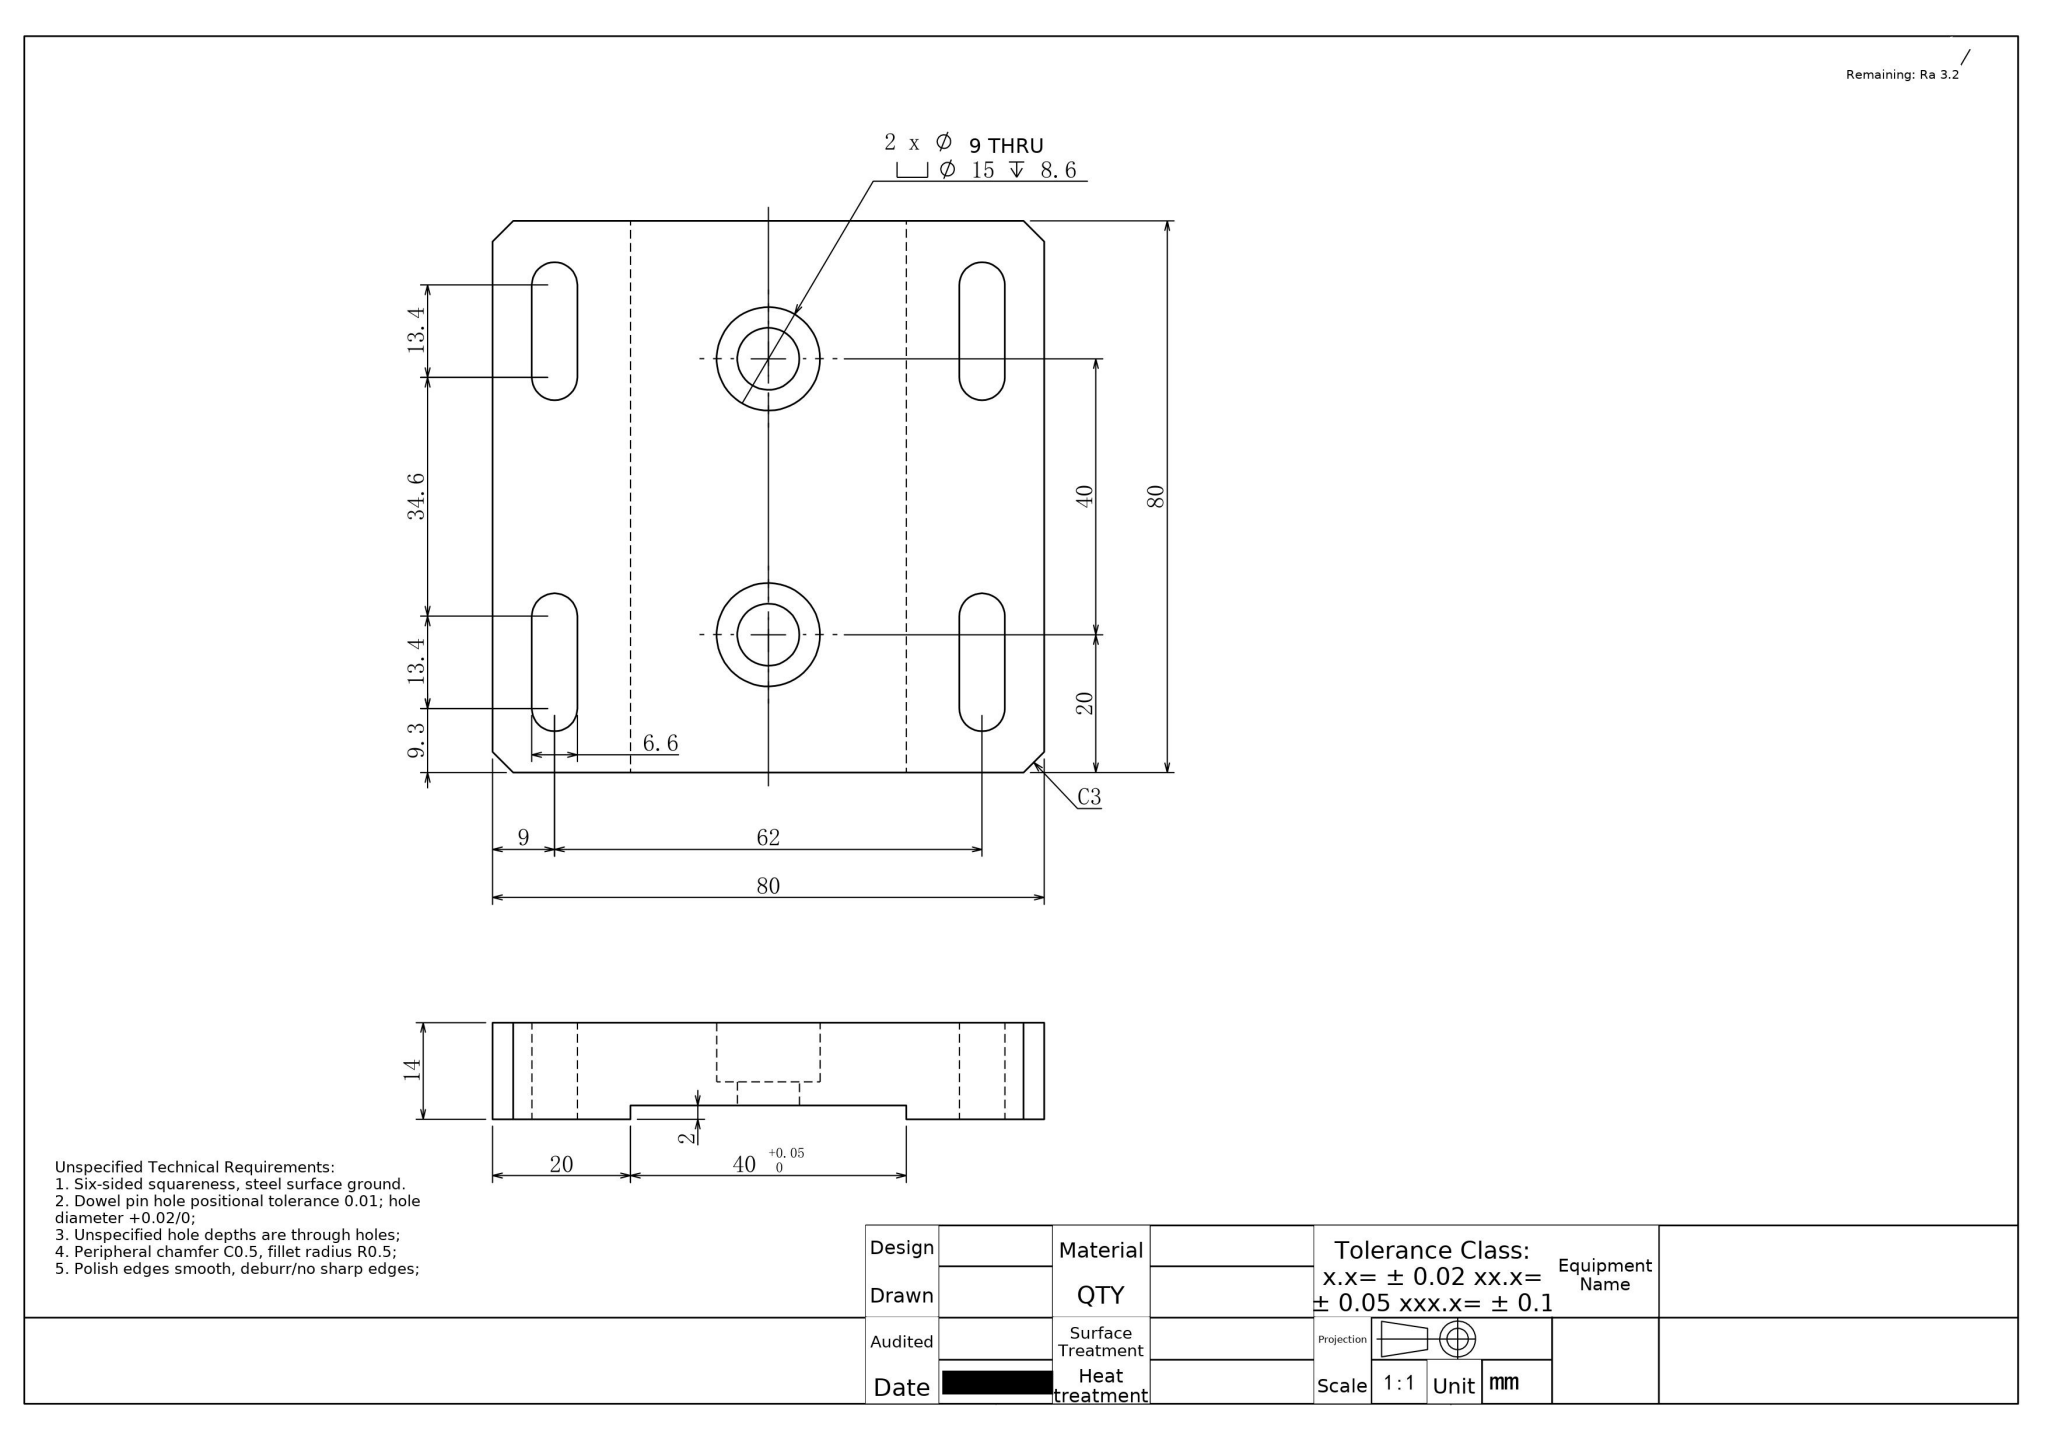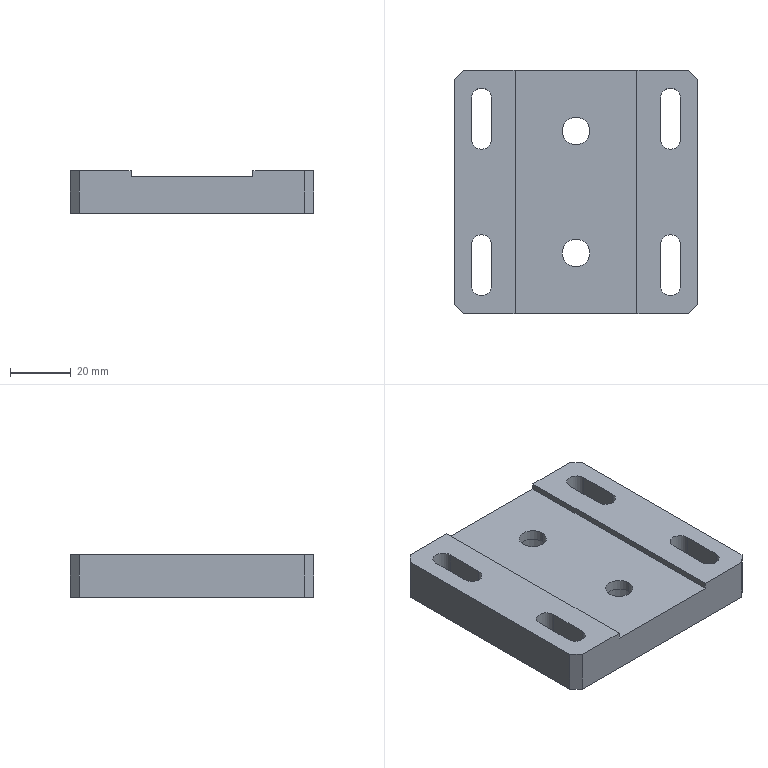Part | NX | mm | 1 solid | 40 faces | box 80 x 80 x 14 mm | volume 72607 mm3 | plane 24 | cylinder 16 | commonest cylinder face diameters 6.6 x8 15 x4 9 x4